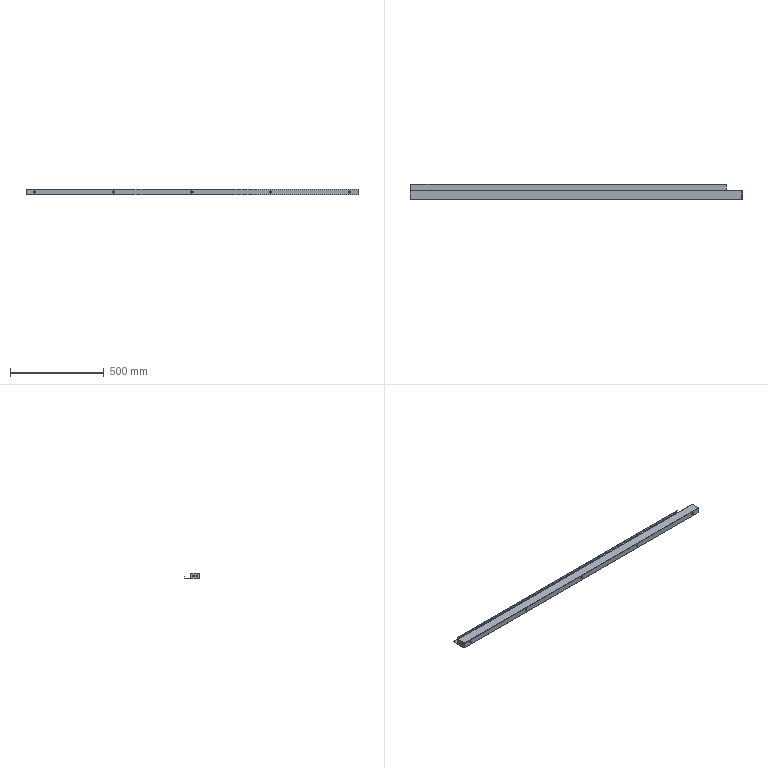Component | SolidWorks | LowerCrossbeam-1 | 1 solid | 84 faces | volume 389371 mm3 | plane 50 | cylinder 34 | commonest cylinder face diameters 11 x14 9 x8 3.4 x6 0.4 x6